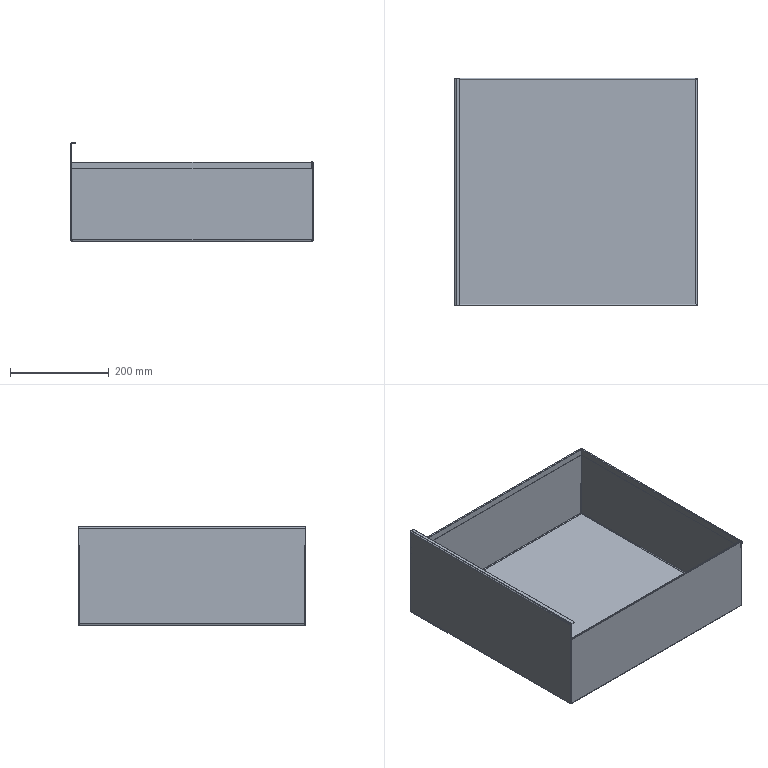Component | SolidWorks | Drawer-1 | 1 solid | 70 faces | volume 852665 mm3 | plane 46 | cylinder 16 | spline 8 | commonest cylinder face diameters 6 x5 3 x5 3.1 x3 0.1 x3